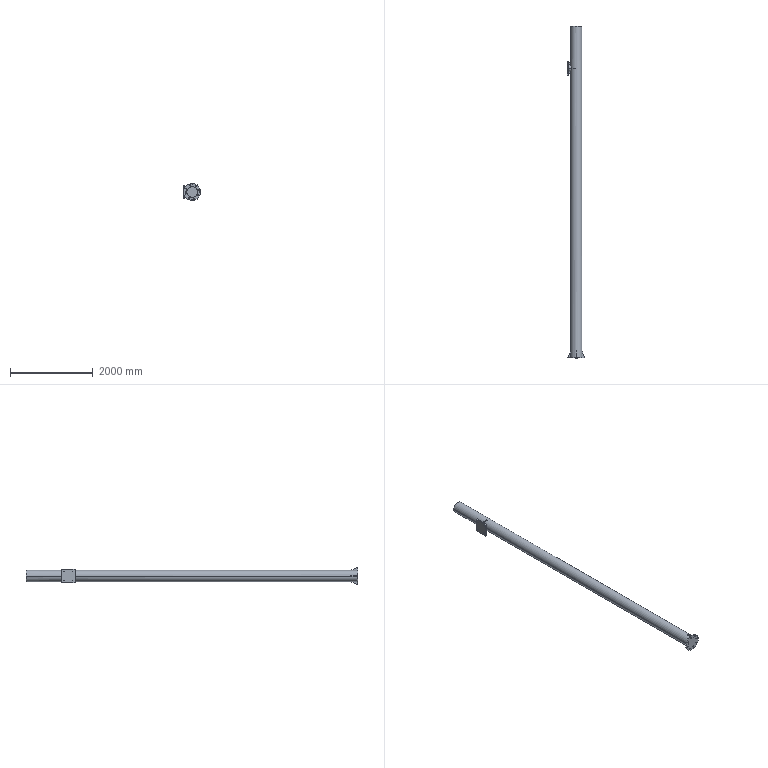Component | SolidWorks | Column-1 | 1 solid | 95 faces | volume 73461058 mm3 | plane 53 | cylinder 34 | cone 8 | commonest cylinder face diameters 24 x16 16 x8 160 x4 413 x2 253 x2 273 x2